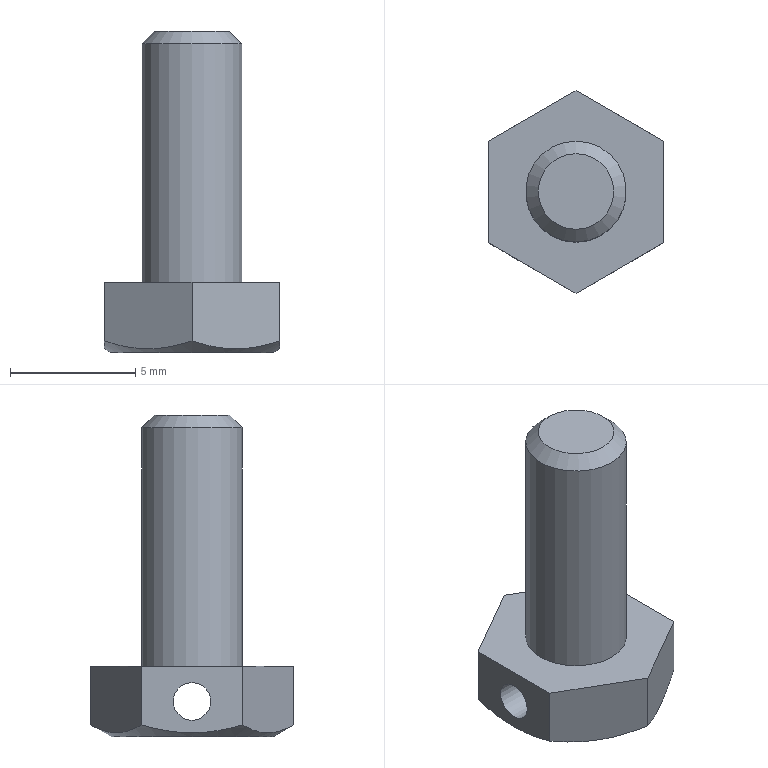Component | NX | BOLT_M4_X_10 | 1 solid | 13 faces | volume 230 mm3 | plane 9 | cylinder 2 | cone 2 | commonest cylinder face diameters 4.013 x1 1.5 x1